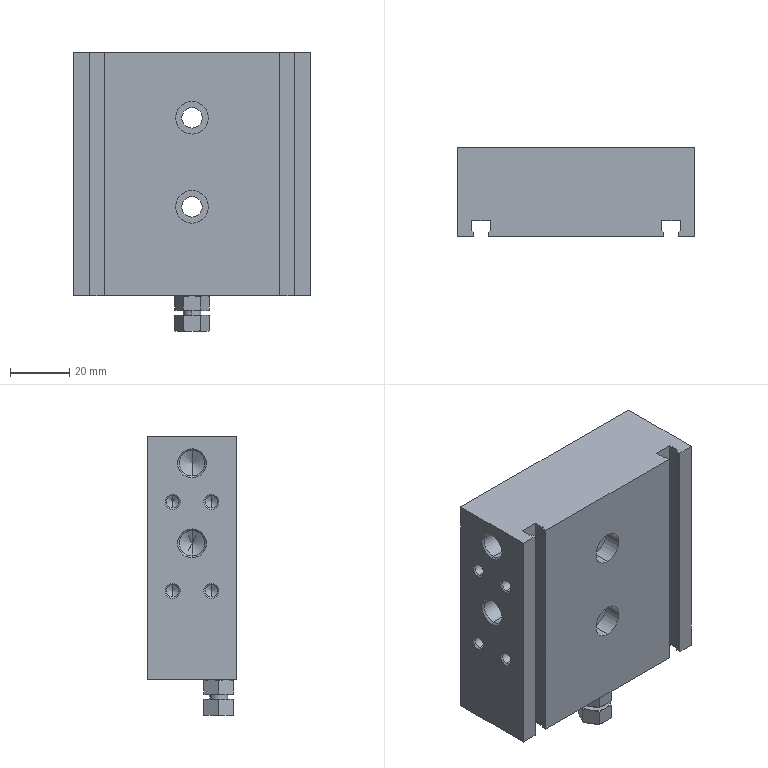Component | SolidWorks | CXSM25-10-Z73(0_0_0)-2_CXSM25-10(0_0)_BODY-1 | 1 solid | 161 faces | box 80 x 30 x 94 mm | volume 165460 mm3 | cone 76 | plane 43 | cylinder 42 | commonest cylinder face diameters 4.134 x16 8.566 x8 11 x4 25 x4 12 x4 6.9 x4 6 x2
build123d program:
from build123d import *

# Parameters (mm, degrees)
BOSS_EXTRUDE1_DEPTH = 82
SKETCH22_R          = 11
CUT_EXTRUDE1_DEPTH  = 12


with BuildPart() as part:
    # Sketch1 → Boss-Extrude1 (new body)
    with BuildSketch(Plane.XY):
        Polygon((-15, 40), (-15, -40), (15, -40), (15, -34.5), (13.575, -34.5), (13.2, -35.15), (9.6, -35.15), (9.6, -28.85), (13.2, -28.85), (13.575, -29.5), (15, -29.5), (15, 29.5), (13.575, 29.5), (13.2, 28.85), (9.6, 28.85), (9.6, 35.15), (13.2, 35.15), (13.575, 34.5), (15, 34.5), (15, 40), align=None)
    extrude(amount=-BOSS_EXTRUDE1_DEPTH)

    # Sketch2 → Cut-Revolve1 (revolve, cut)
    with BuildSketch(Plane(origin=(0, 0, 0), x_dir=(0, 0, -1), z_dir=(1, 0, 0)), mode=Mode.PRIVATE) as cut_revolve1_sk:
        Polygon((0, 17.5), (0, 23.5), (30, 23.5), (30, 30), (45, 30), (45, 17.5), align=None)
    revolve(cut_revolve1_sk.sketch.rotate(Axis((0, 17.5, -45), (0, 0, 1)), 270), axis=Axis((0, 17.5, -45), (0, 0, 1)), mode=Mode.SUBTRACT)

    # Sketch3 → Cut-Revolve2 (revolve, cut)
    with BuildSketch(Plane(origin=(0, 0, 0), x_dir=(0, 0, -1), z_dir=(1, 0, 0)), mode=Mode.PRIVATE) as cut_revolve2_sk:
        Polygon((0, -17.5), (0, -11.5), (30, -11.5), (30, -5), (45, -5), (45, -17.5), align=None)
    revolve(cut_revolve2_sk.sketch.rotate(Axis((0, -17.5, -45), (0, 0, 1)), 270), axis=Axis((0, -17.5, -45), (0, 0, 1)), mode=Mode.SUBTRACT)

    # Sketch4 → Cut-Revolve3 (revolve, cut)
    with BuildSketch(Plane.XY.offset(-30), mode=Mode.PRIVATE) as cut_revolve3_sk:
        Polygon((-15, 0), (-15, 3.45), (8.7, 3.45), (8.7, 5.5), (15, 5.5), (15, 0), align=None)
    revolve(cut_revolve3_sk.sketch.rotate(Axis((15, 0, -30), (-1, 0, 0)), 270), axis=Axis((15, 0, -30), (-1, 0, 0)), mode=Mode.SUBTRACT)

    # Sketch5 → Cut-Revolve4 (revolve, cut)
    with BuildSketch(Plane.XY.offset(-60), mode=Mode.PRIVATE) as cut_revolve4_sk:
        Polygon((-15, 0), (-15, 3.45), (8.7, 3.45), (8.7, 5.5), (15, 5.5), (15, 0), align=None)
    revolve(cut_revolve4_sk.sketch.rotate(Axis((15, 0, -60), (-1, 0, 0)), 270), axis=Axis((15, 0, -60), (-1, 0, 0)), mode=Mode.SUBTRACT)

    # Sketch6 → Cut-Revolve5 (revolve, cut)
    with BuildSketch(Plane.XY.offset(-30), mode=Mode.PRIVATE) as cut_revolve5_sk:
        Polygon((-15, 0), (-15, 4), (-14.323, 3.324), (-3, 3.324), (-1.081, 0), align=None)
    revolve(cut_revolve5_sk.sketch.rotate(Axis((-1.081, 0, -30), (-1, 0, 0)), 270), axis=Axis((-1.081, 0, -30), (-1, 0, 0)), mode=Mode.SUBTRACT)

    # Sketch7 → Cut-Revolve6 (revolve, cut)
    with BuildSketch(Plane.XY.offset(-60), mode=Mode.PRIVATE) as cut_revolve6_sk:
        Polygon((-15, 0), (-15, 4), (-14.323, 3.324), (-3, 3.324), (-1.081, 0), align=None)
    revolve(cut_revolve6_sk.sketch.rotate(Axis((-1.081, 0, -60), (-1, 0, 0)), 270), axis=Axis((-1.081, 0, -60), (-1, 0, 0)), mode=Mode.SUBTRACT)

    # Sketch8 → Cut-Revolve7 (revolve, cut)
    with BuildSketch(Plane.XY.offset(-30), mode=Mode.PRIVATE) as cut_revolve7_sk:
        Polygon((-6.5, 31.307), (-8.567, 32.5), (-8.567, 39.567), (-9, 40), (-6.5, 40), align=None)
    revolve(cut_revolve7_sk.sketch.rotate(Axis((-6.5, 40, -30), (0, -1, 0)), 90), axis=Axis((-6.5, 40, -30), (0, -1, 0)), mode=Mode.SUBTRACT)

    # Sketch9 → Cut-Revolve8 (revolve, cut)
    with BuildSketch(Plane.XY.offset(-30), mode=Mode.PRIVATE) as cut_revolve8_sk:
        Polygon((6.5, -40), (4, -40), (4.433, -39.567), (4.433, -32.5), (6.5, -31.307), align=None)
    revolve(cut_revolve8_sk.sketch.rotate(Axis((6.5, -31.307, -30), (0, -1, 0)), 90), axis=Axis((6.5, -31.307, -30), (0, -1, 0)), mode=Mode.SUBTRACT)

    # Sketch10 → Cut-Revolve9 (revolve, cut)
    with BuildSketch(Plane(origin=(0, 0, 0), x_dir=(0, 0, -1), z_dir=(1, 0, 0)), mode=Mode.PRIVATE) as cut_revolve9_sk:
        Polygon((46, 31.027), (41.717, 33.5), (41.717, 39.419), (41.136, 40), (46, 40), align=None)
    revolve(cut_revolve9_sk.sketch.rotate(Axis((0, 40, -46), (0, -1, 0)), 180), axis=Axis((0, 40, -46), (0, -1, 0)), mode=Mode.SUBTRACT)

    # Sketch11 → Cut-Revolve10 (revolve, cut)
    with BuildSketch(Plane(origin=(0, 0, 0), x_dir=(0, 0, -1), z_dir=(1, 0, 0)), mode=Mode.PRIVATE) as cut_revolve10_sk:
        Polygon((73, 31.027), (68.717, 33.5), (68.717, 39.419), (68.136, 40), (73, 40), align=None)
    revolve(cut_revolve10_sk.sketch.rotate(Axis((0, 40, -73), (0, -1, 0)), 180), axis=Axis((0, 40, -73), (0, -1, 0)), mode=Mode.SUBTRACT)

    # Sketch12 → Cut-Revolve11 (revolve, cut)
    with BuildSketch(Plane(origin=(0, 0, 0), x_dir=(0, 0, -1), z_dir=(1, 0, 0)), mode=Mode.PRIVATE) as cut_revolve11_sk:
        Polygon((46, -40), (41.136, -40), (41.717, -39.419), (41.717, -33.5), (46, -31.027), align=None)
    revolve(cut_revolve11_sk.sketch.rotate(Axis((0, -31.027, -46), (0, -1, 0)), 180), axis=Axis((0, -31.027, -46), (0, -1, 0)), mode=Mode.SUBTRACT)

    # Sketch13 → Cut-Revolve12 (revolve, cut)
    with BuildSketch(Plane(origin=(0, 0, 0), x_dir=(0, 0, -1), z_dir=(1, 0, 0)), mode=Mode.PRIVATE) as cut_revolve12_sk:
        Polygon((73, -40), (68.136, -40), (68.717, -39.419), (68.717, -33.5), (73, -31.027), align=None)
    revolve(cut_revolve12_sk.sketch.rotate(Axis((0, -31.027, -73), (0, -1, 0)), 180), axis=Axis((0, -31.027, -73), (0, -1, 0)), mode=Mode.SUBTRACT)

    # Sketch14 → Cut-Revolve13 (revolve, cut)
    with BuildSketch(Plane.XY.offset(-60), mode=Mode.PRIVATE) as cut_revolve13_sk:
        Polygon((6.5, 31.307), (4.433, 32.5), (4.433, 39.567), (4, 40), (6.5, 40), align=None)
    revolve(cut_revolve13_sk.sketch.rotate(Axis((6.5, 40, -60), (0, -1, 0)), 90), axis=Axis((6.5, 40, -60), (0, -1, 0)), mode=Mode.SUBTRACT)

    # Sketch15 → Cut-Revolve14 (revolve, cut)
    with BuildSketch(Plane.XY.offset(-60), mode=Mode.PRIVATE) as cut_revolve14_sk:
        Polygon((-6.5, 31.307), (-8.567, 32.5), (-8.567, 39.567), (-9, 40), (-6.5, 40), align=None)
    revolve(cut_revolve14_sk.sketch.rotate(Axis((-6.5, 40, -60), (0, -1, 0)), 90), axis=Axis((-6.5, 40, -60), (0, -1, 0)), mode=Mode.SUBTRACT)

    # Sketch16 → Cut-Revolve15 (revolve, cut)
    with BuildSketch(Plane.XY.offset(-30), mode=Mode.PRIVATE) as cut_revolve15_sk:
        Polygon((6.5, 31.307), (4.433, 32.5), (4.433, 39.567), (4, 40), (6.5, 40), align=None)
    revolve(cut_revolve15_sk.sketch.rotate(Axis((6.5, 40, -30), (0, -1, 0)), 90), axis=Axis((6.5, 40, -30), (0, -1, 0)), mode=Mode.SUBTRACT)

    # Sketch17 → Cut-Revolve16 (revolve, cut)
    with BuildSketch(Plane.XY.offset(-60), mode=Mode.PRIVATE) as cut_revolve16_sk:
        Polygon((-6.5, -40), (-9, -40), (-8.567, -39.567), (-8.567, -32.5), (-6.5, -31.307), align=None)
    revolve(cut_revolve16_sk.sketch.rotate(Axis((-6.5, -31.307, -60), (0, -1, 0)), 90), axis=Axis((-6.5, -31.307, -60), (0, -1, 0)), mode=Mode.SUBTRACT)

    # Sketch18 → Cut-Revolve17 (revolve, cut)
    with BuildSketch(Plane.XY.offset(-60), mode=Mode.PRIVATE) as cut_revolve17_sk:
        Polygon((6.5, -40), (4, -40), (4.433, -39.567), (4.433, -32.5), (6.5, -31.307), align=None)
    revolve(cut_revolve17_sk.sketch.rotate(Axis((6.5, -31.307, -60), (0, -1, 0)), 90), axis=Axis((6.5, -31.307, -60), (0, -1, 0)), mode=Mode.SUBTRACT)

    # Sketch19 → Cut-Revolve18 (revolve, cut)
    with BuildSketch(Plane.XY.offset(-30), mode=Mode.PRIVATE) as cut_revolve18_sk:
        Polygon((-6.5, -40), (-9, -40), (-8.567, -39.567), (-8.567, -32.5), (-6.5, -31.307), align=None)
    revolve(cut_revolve18_sk.sketch.rotate(Axis((-6.5, -31.307, -30), (0, -1, 0)), 90), axis=Axis((-6.5, -31.307, -30), (0, -1, 0)), mode=Mode.SUBTRACT)

    # Sketch20 → Revolve1 (revolve)
    with BuildSketch(Plane(origin=(9, 0, 0), x_dir=(0, 0, -1), z_dir=(1, 0, 0)), mode=Mode.PRIVATE) as revolve1_sk:
        Polygon((-5, 0), (-5, 5), (-3.66, 10), (-1.34, 10), (0, 5), (0, 0), align=None)
    revolve(revolve1_sk.sketch.rotate(Axis((9, 0, 0), (0, 0, 1)), 270), axis=Axis((9, 0, 0), (0, 0, 1)))

    # Sketch21 → Revolve2 (revolve)
    with BuildSketch(Plane(origin=(9, 0, 0), x_dir=(0, 0, -1), z_dir=(1, 0, 0)), mode=Mode.PRIVATE) as revolve2_sk:
        Polygon((-12, 0), (-12, 5), (-10.66, 10), (-7.84, 10), (-6.5, 5), (-6.5, 3), (-5, 3), (-5, 0), align=None)
    revolve(revolve2_sk.sketch.rotate(Axis((9, 0, 5), (0, 0, 1)), 270), axis=Axis((9, 0, 5), (0, 0, 1)))

    # Sketch22 → Cut-Extrude1 (cut)
    with BuildSketch(Plane.XY):
        with Locations((9, 0)):
            Circle(SKETCH22_R)
        Polygon((4, 2.887), (4, -2.887), (9, -5.774), (14, -2.887), (14, 2.887), (9, 5.774), align=None, mode=Mode.SUBTRACT)
    extrude(amount=CUT_EXTRUDE1_DEPTH, mode=Mode.SUBTRACT)


solid = part.part

# Placed as in the assembly
solid = solid.moved(Location((955.268, 376.143, -246.265), (180, 0, 90)))